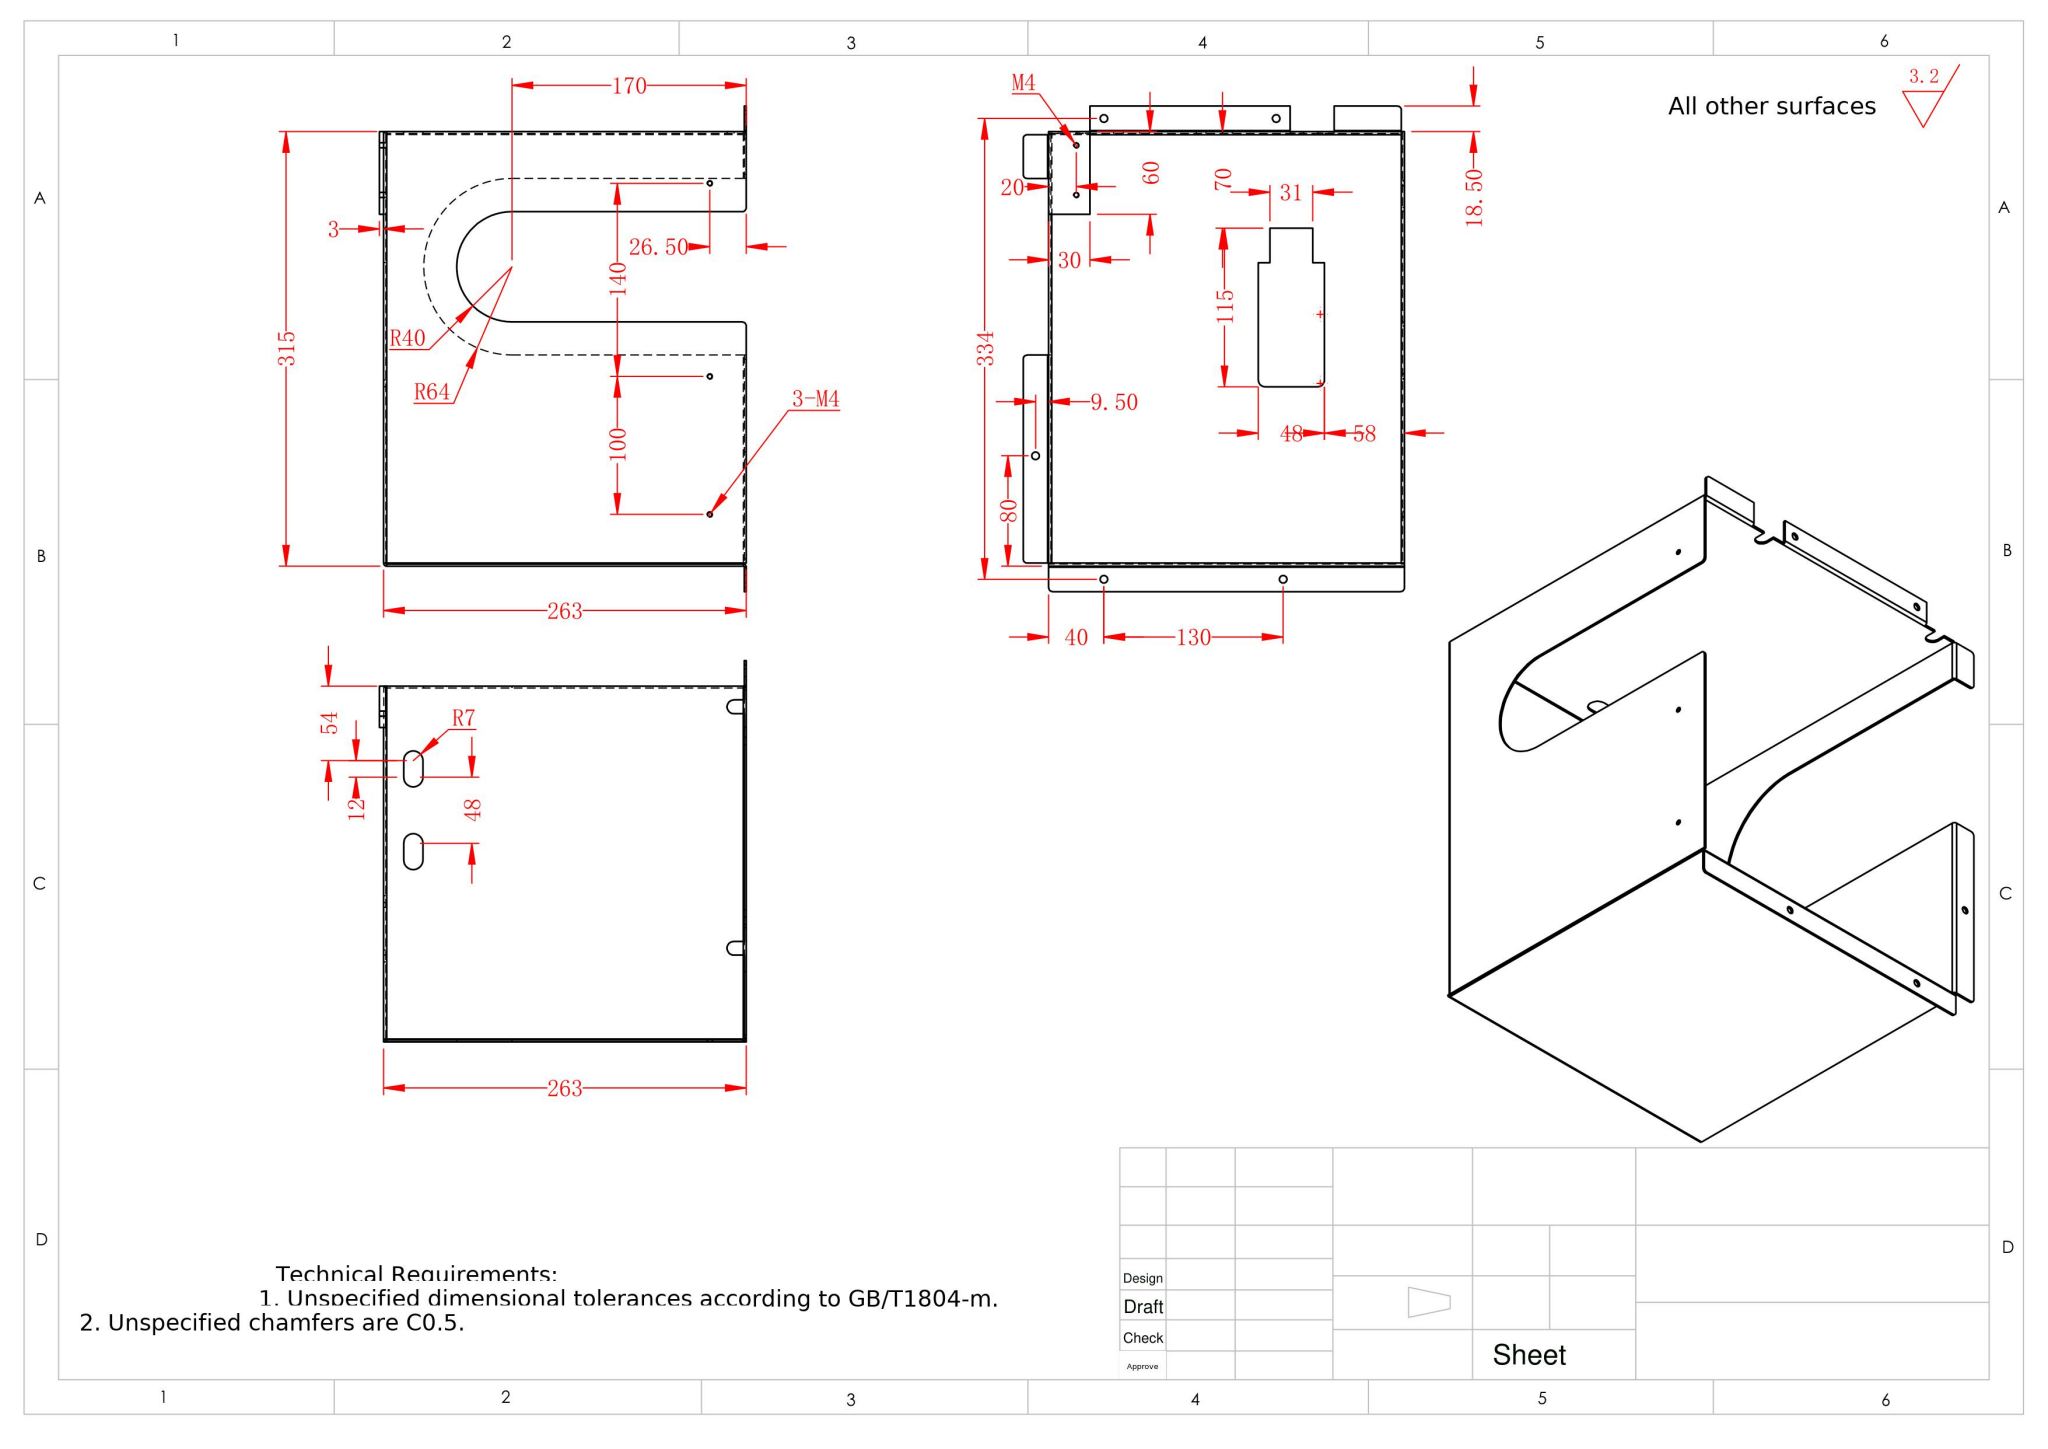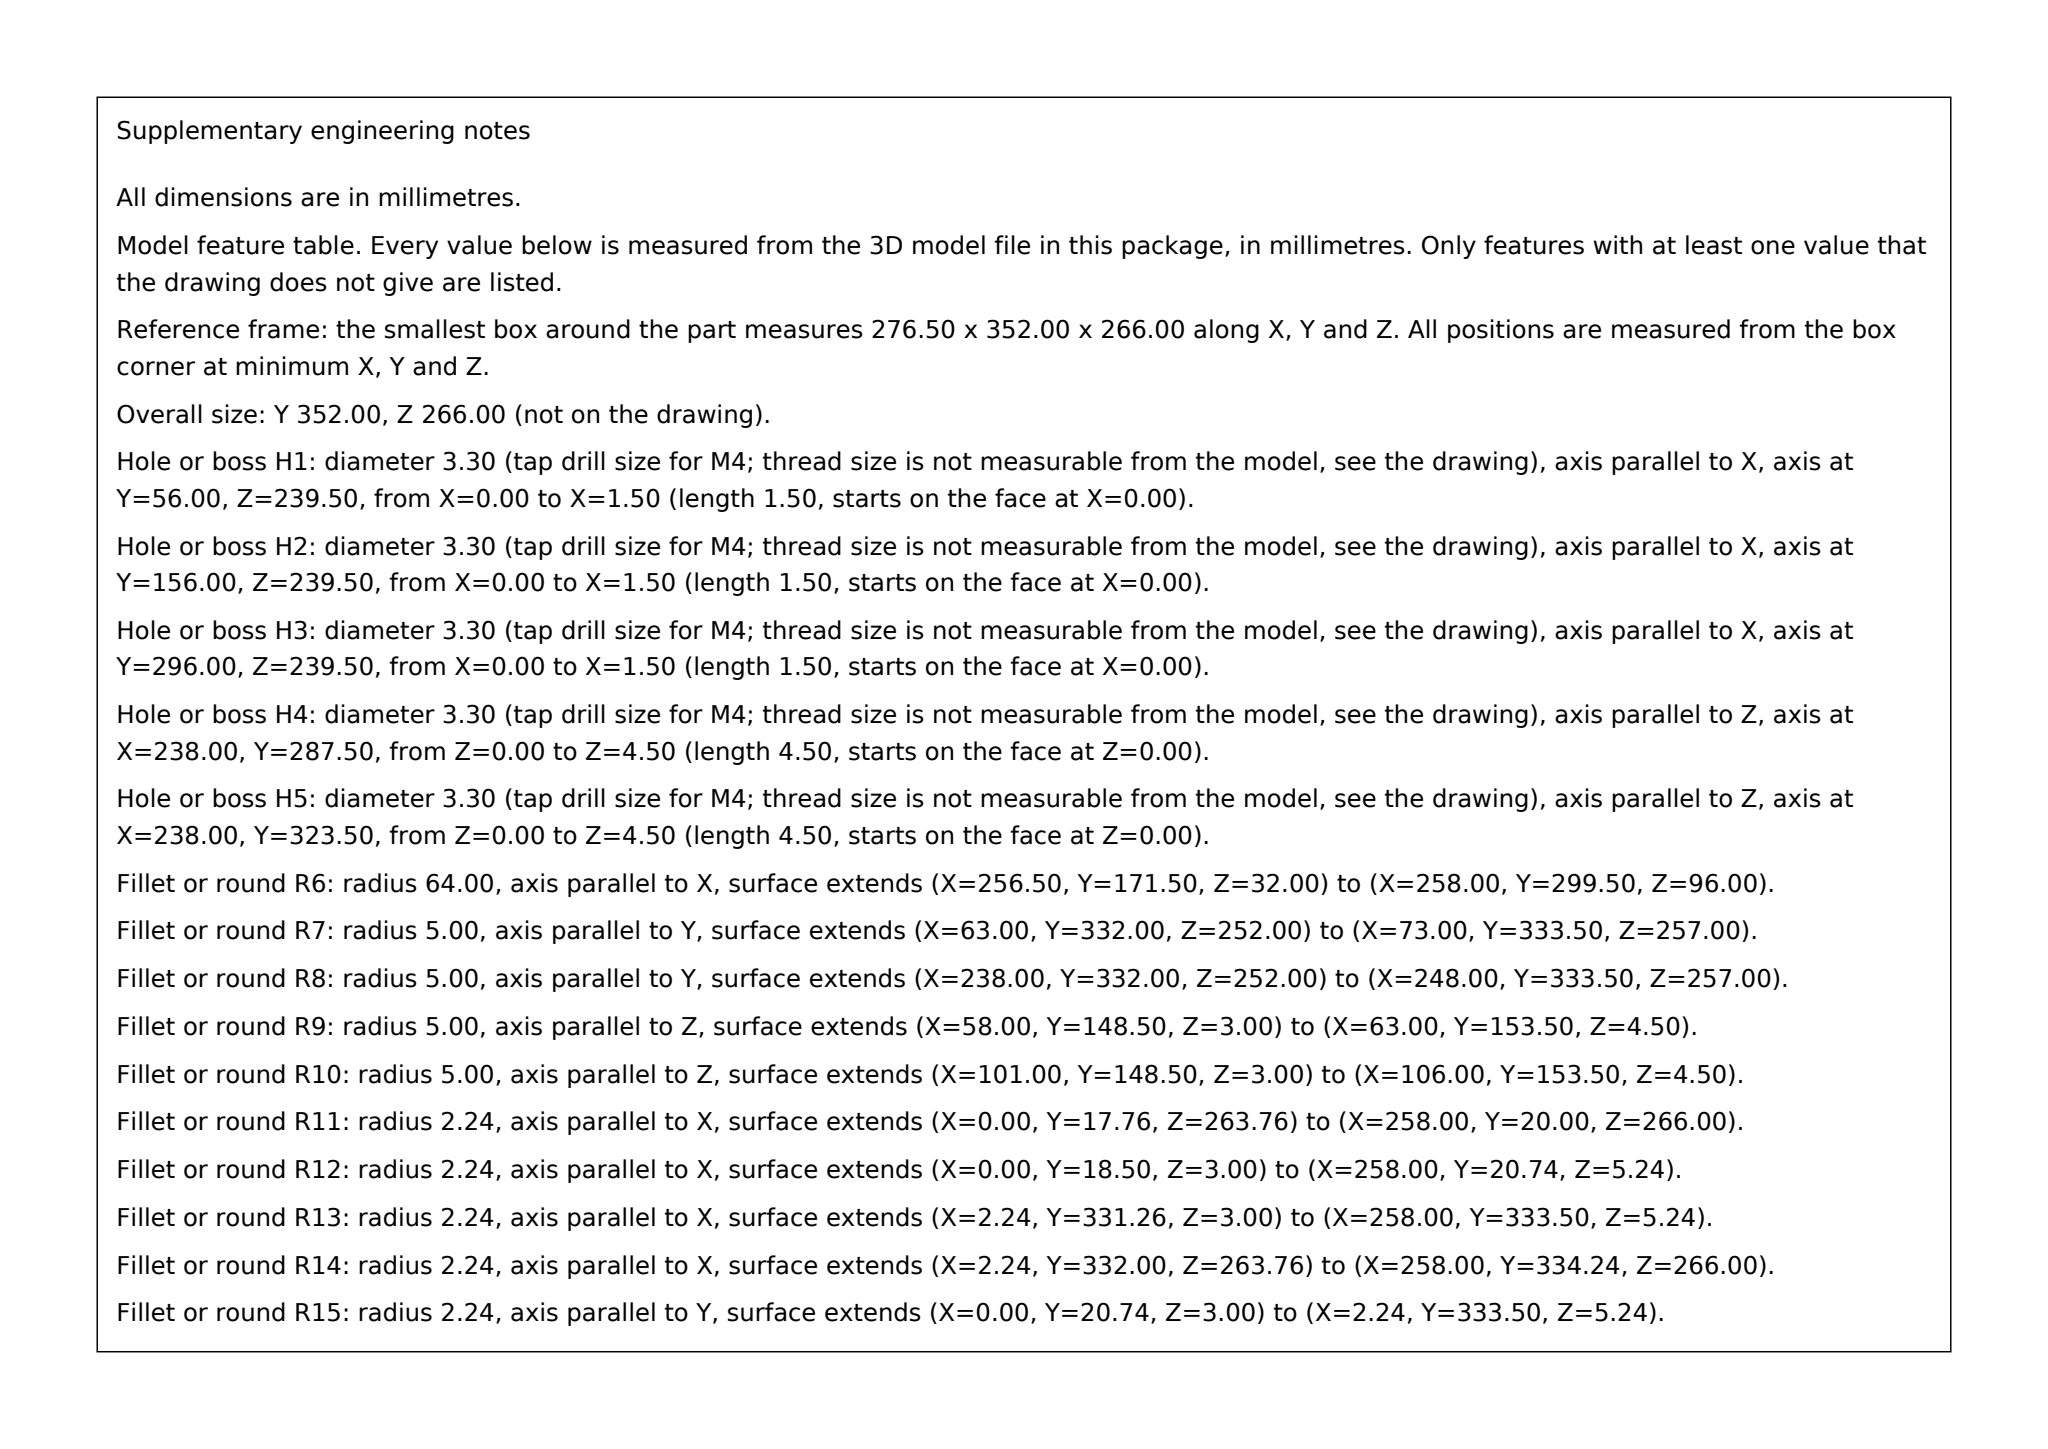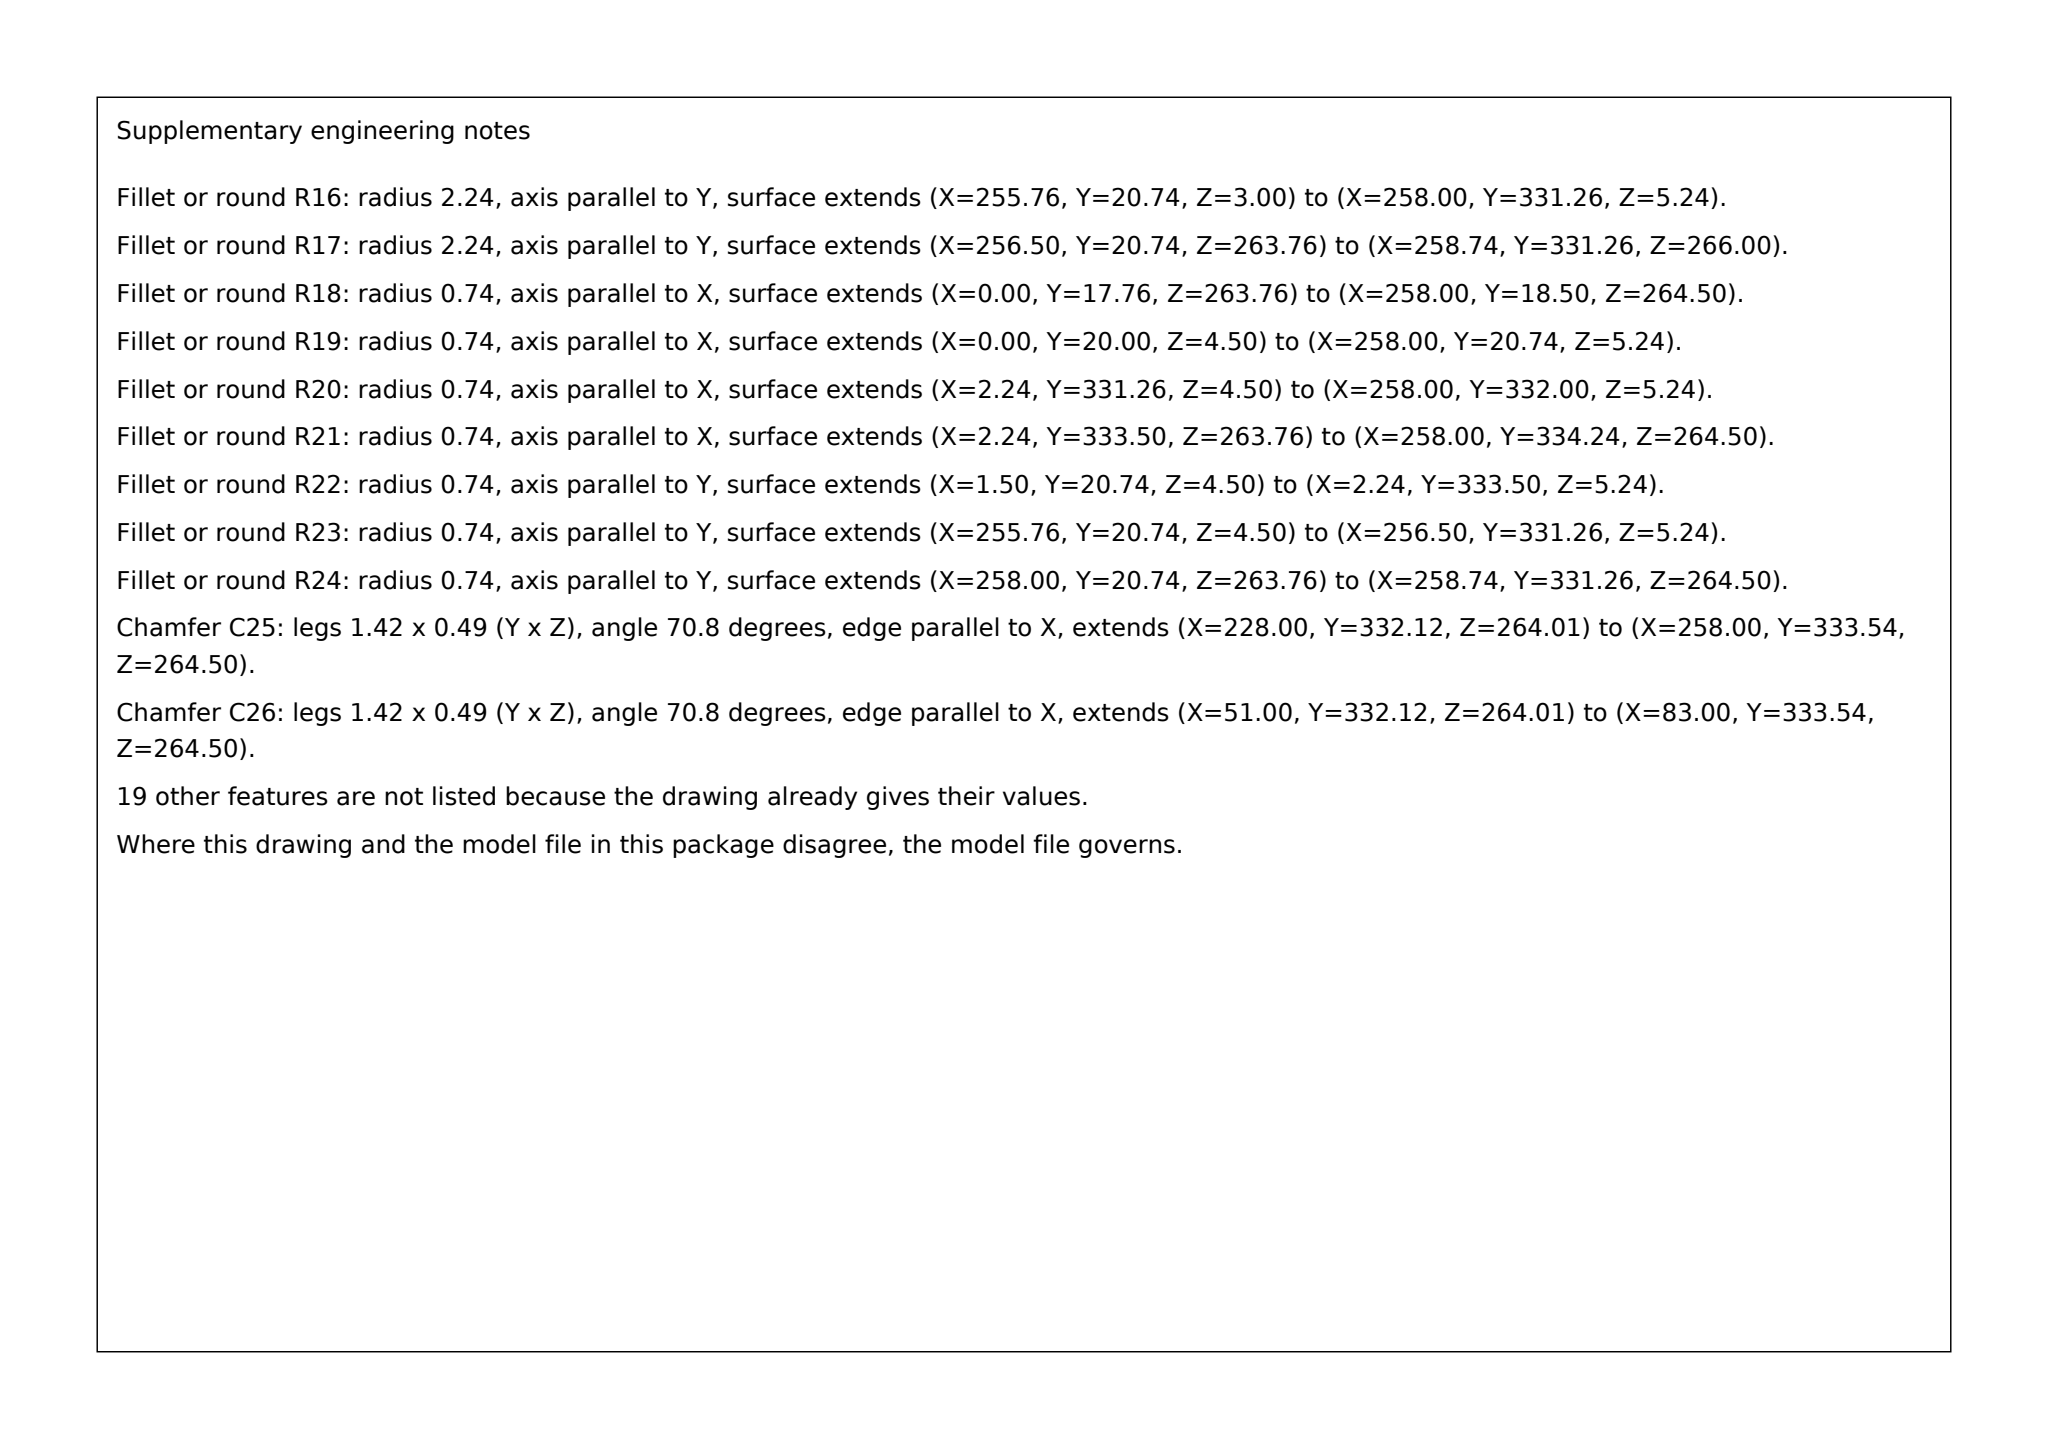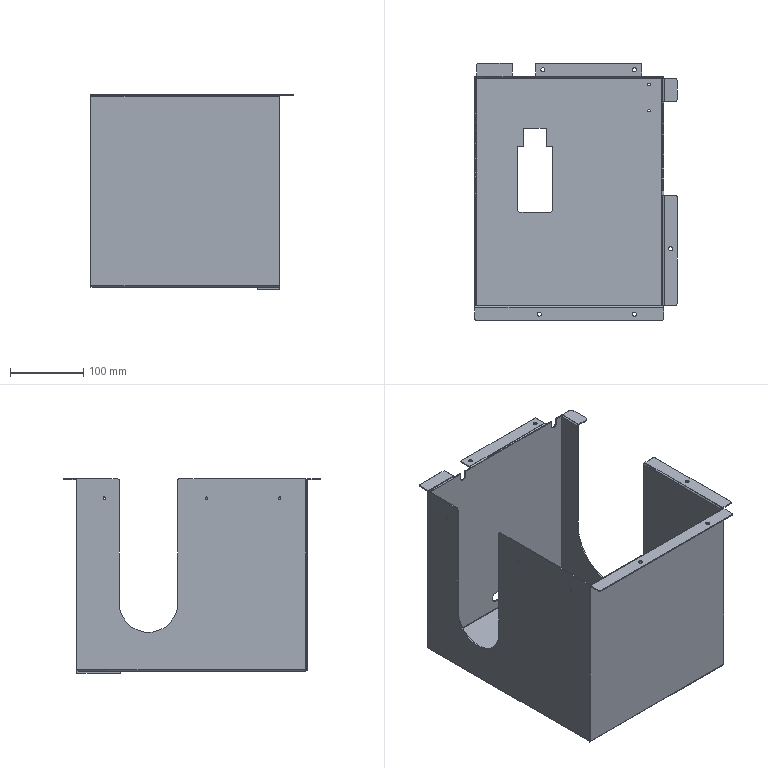Part | SolidWorks | mm | 1 solid | 163 faces | box 276.5 x 352 x 266 mm | volume 513442 mm3 | plane 101 | cylinder 62 | commonest cylinder face diameters 3.3 x10 5.5 x10 4.473 x10 1.473 x10 6 x9 10 x6 14 x4 128 x2